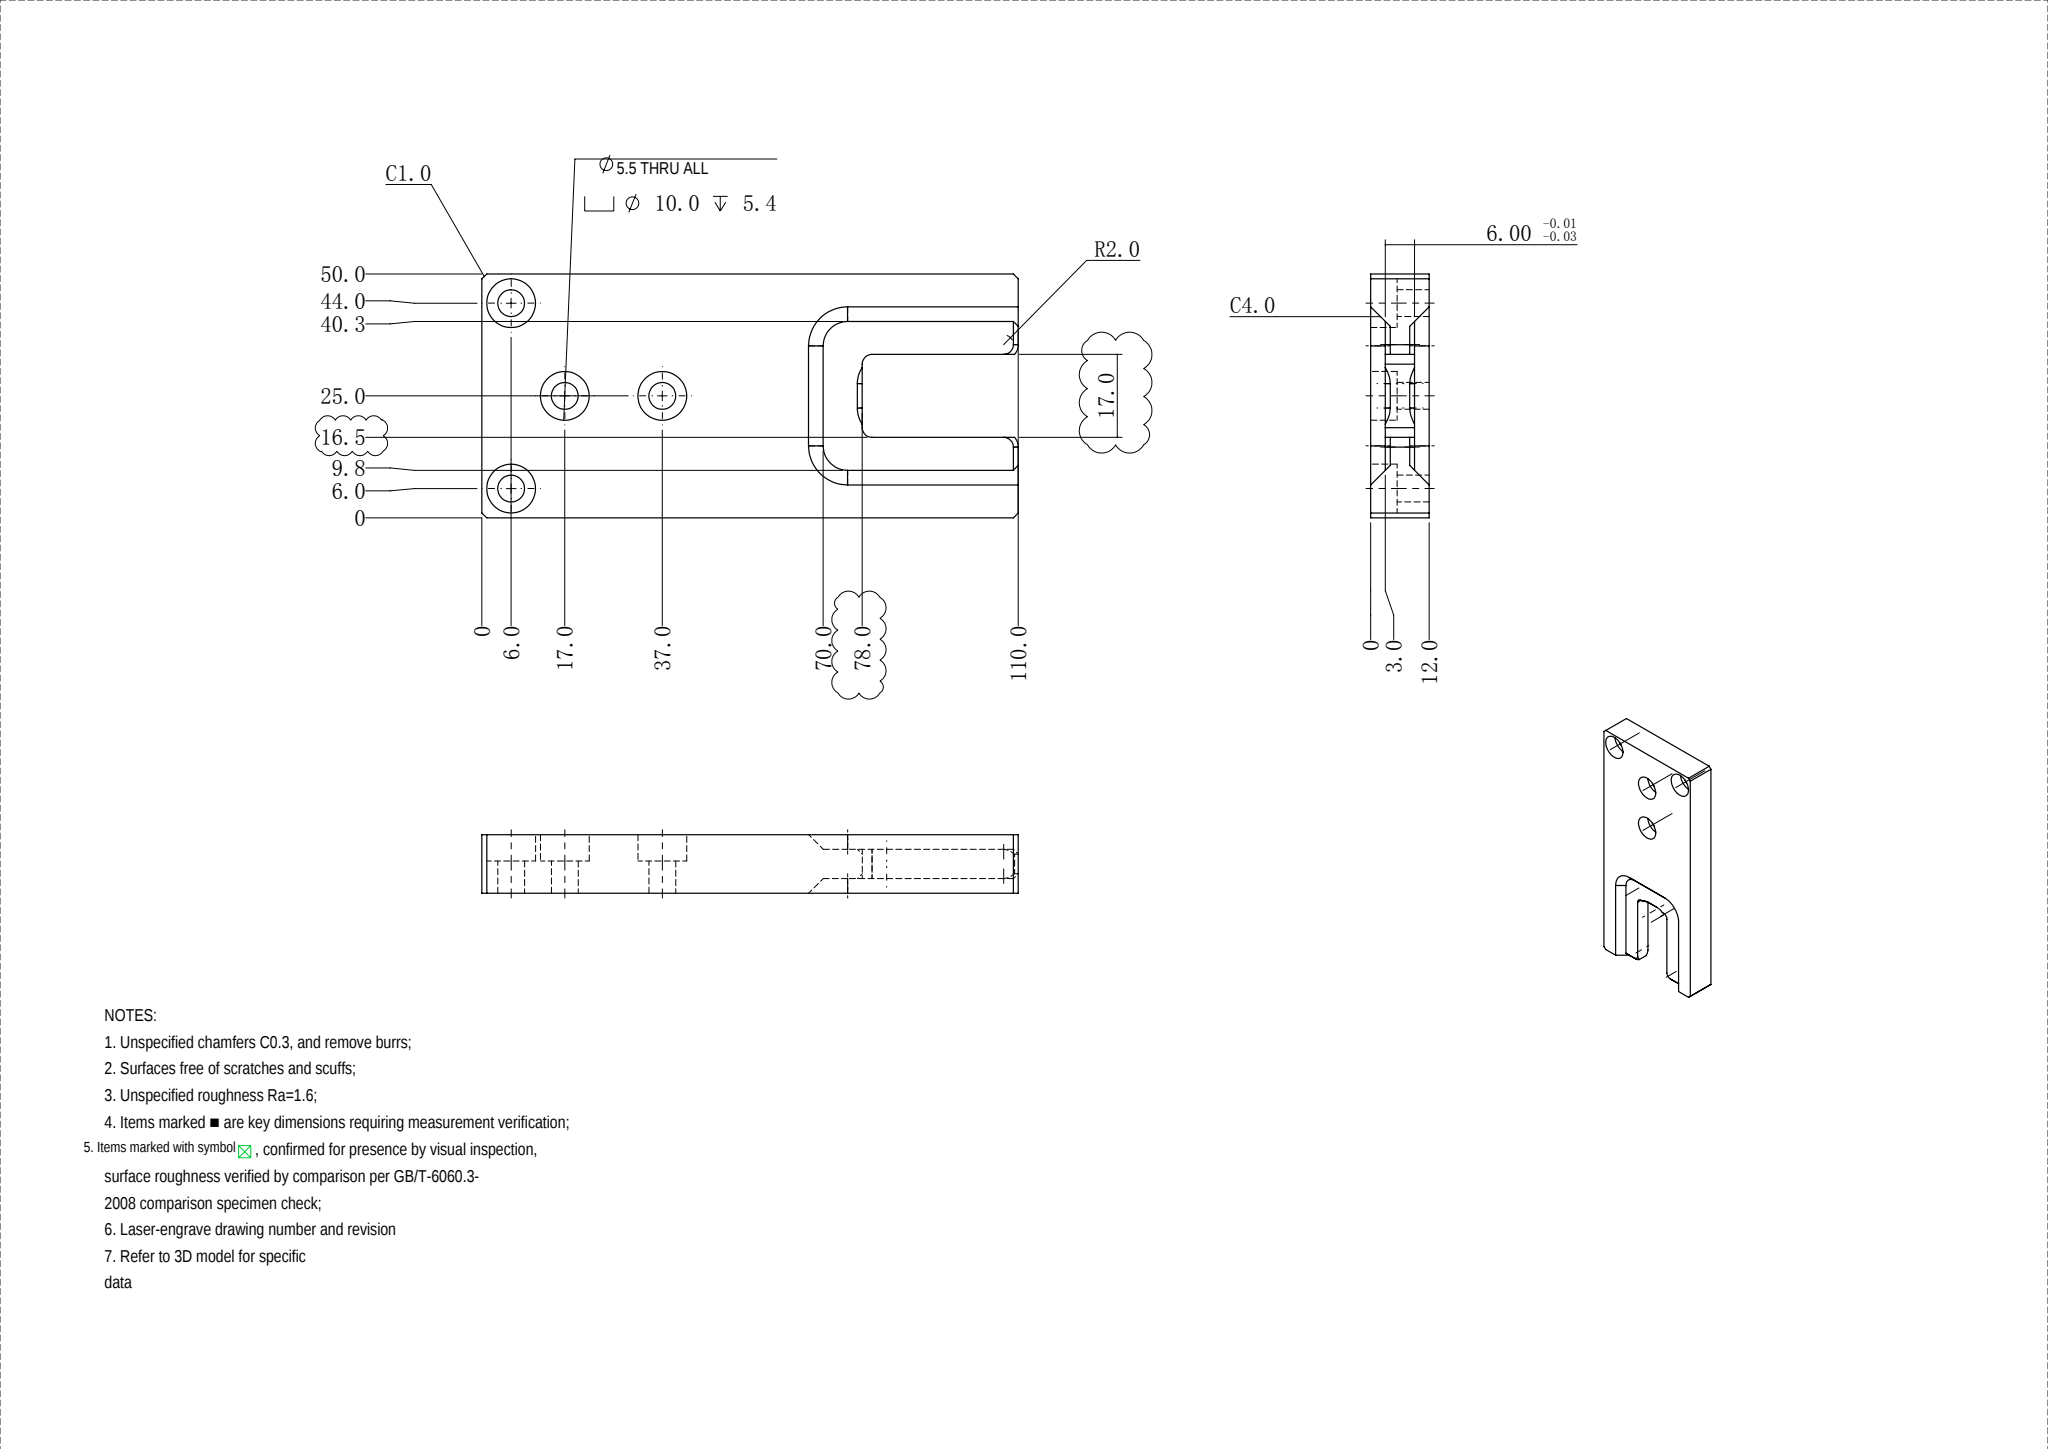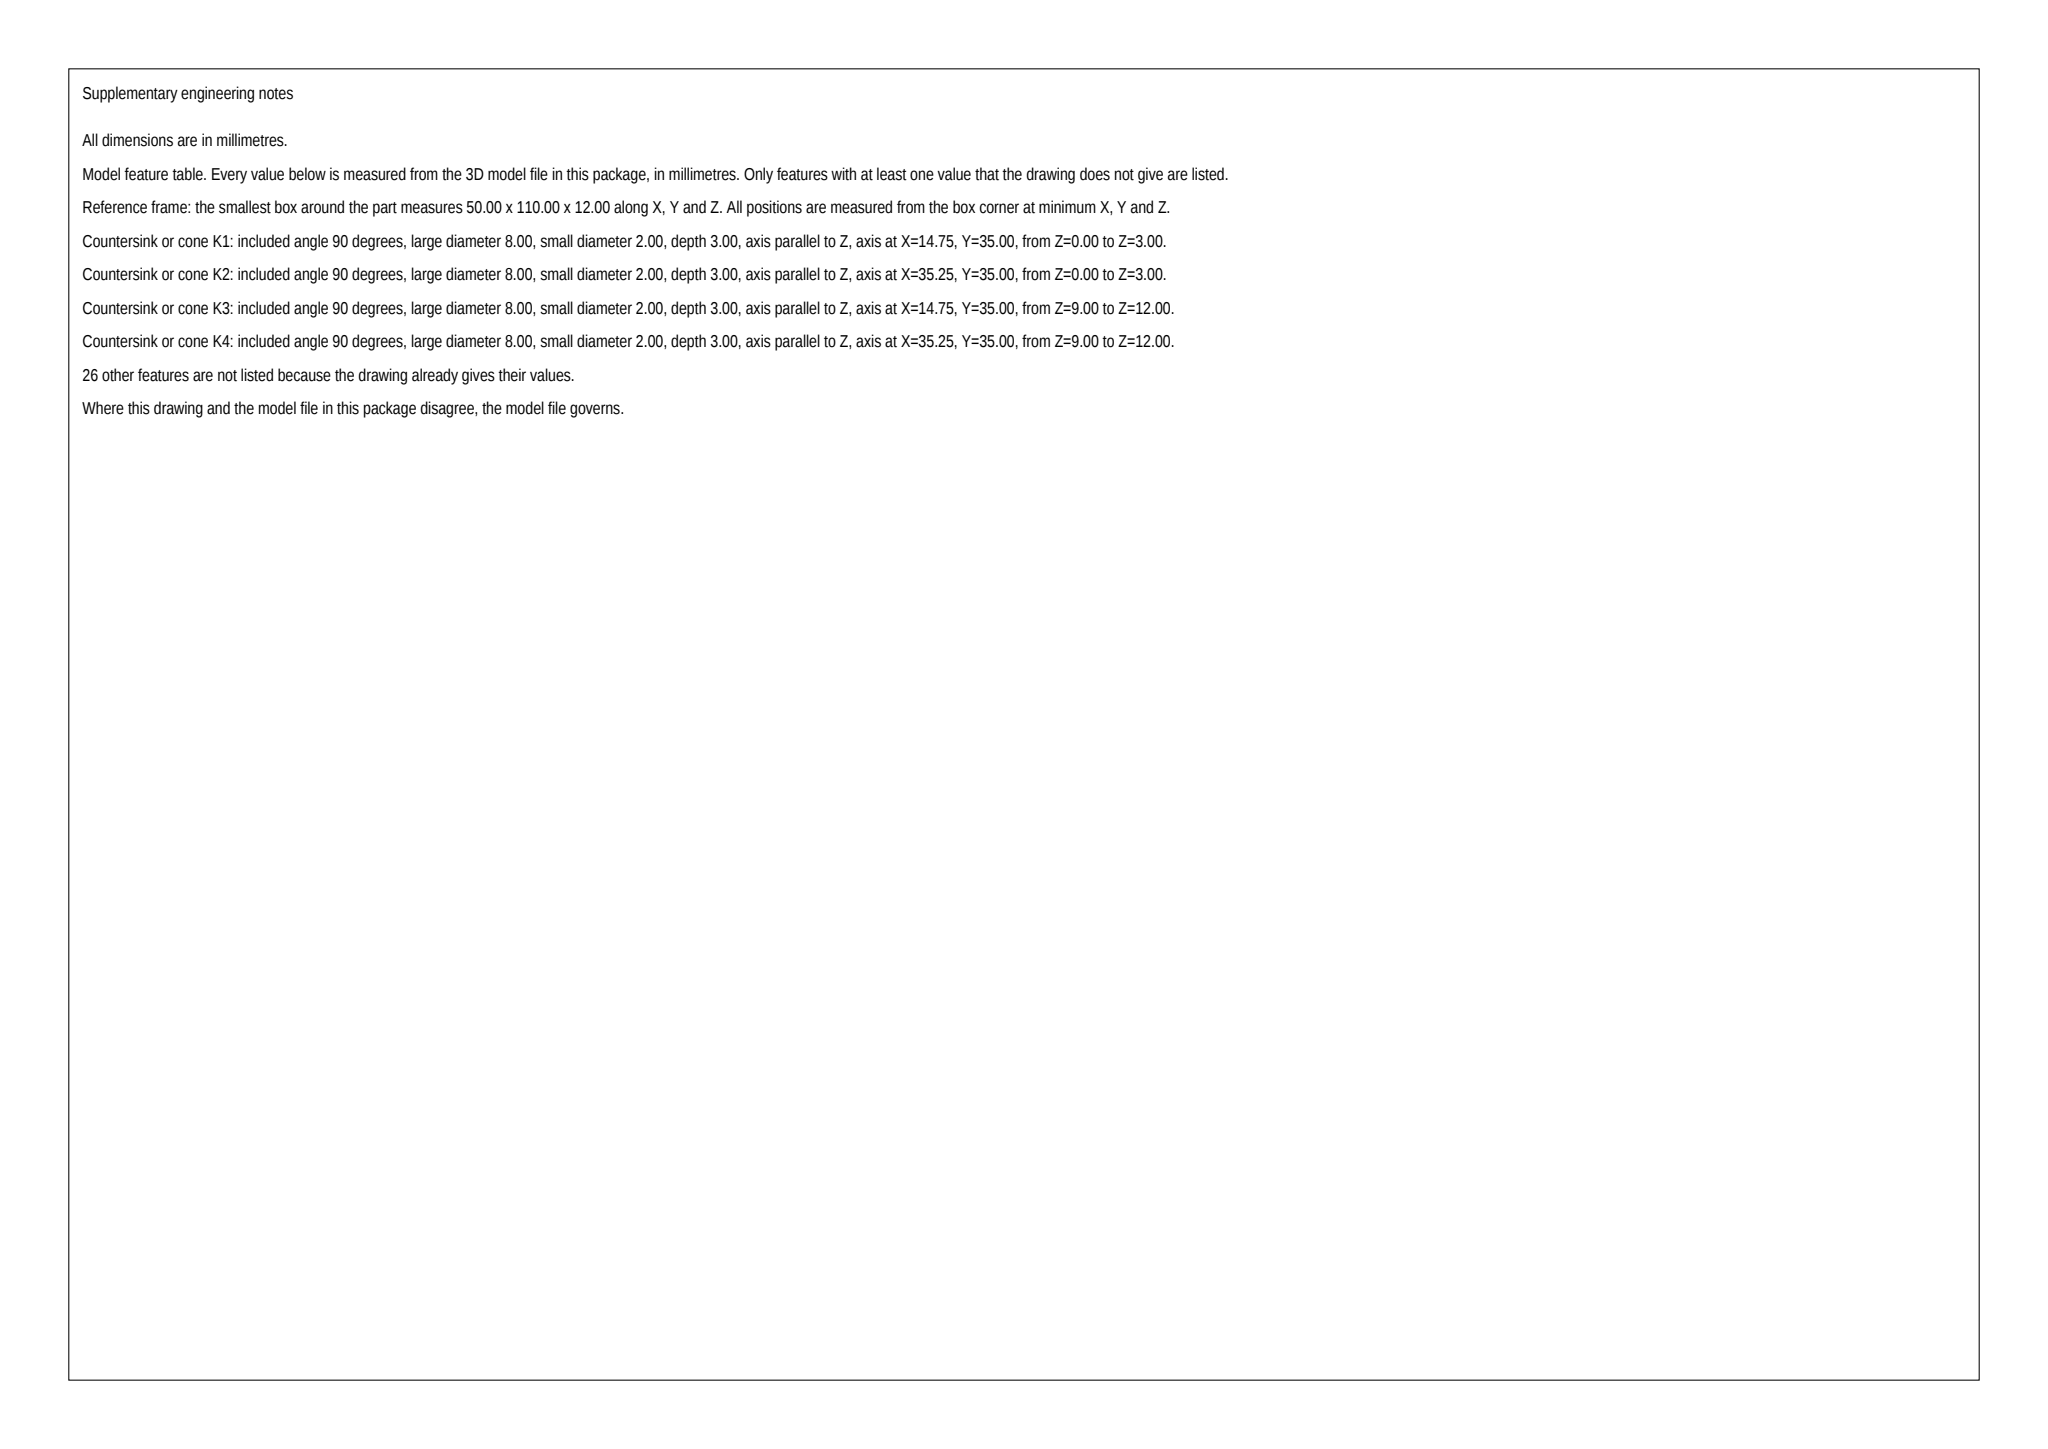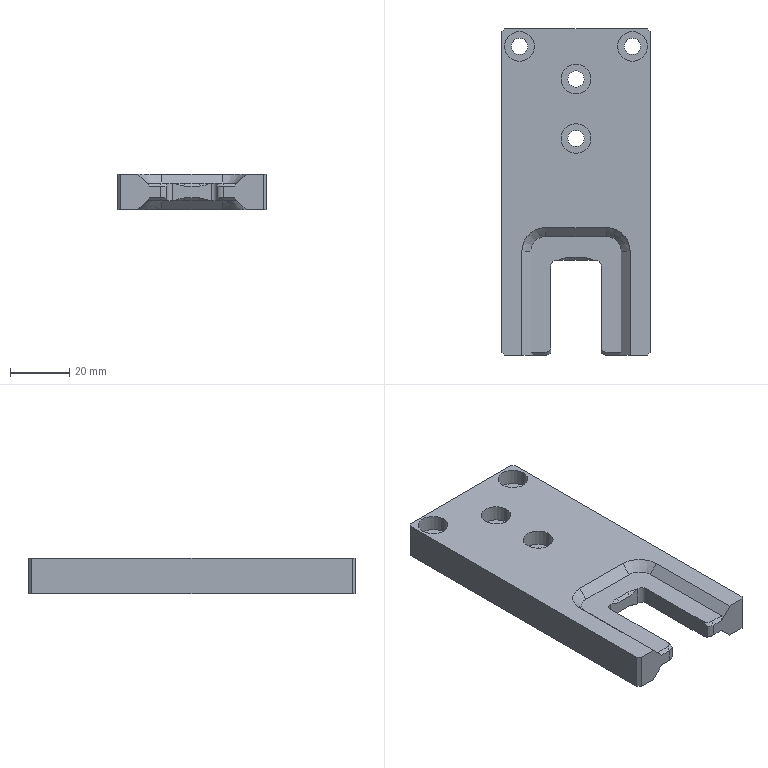Part | SolidWorks | mm | 1 solid | 64 faces | box 50 x 110 x 12 mm | volume 52131 mm3 | plane 32 | cylinder 20 | cone 12 | commonest cylinder face diameters 10 x8 5.5 x8 6 x2 4 x2